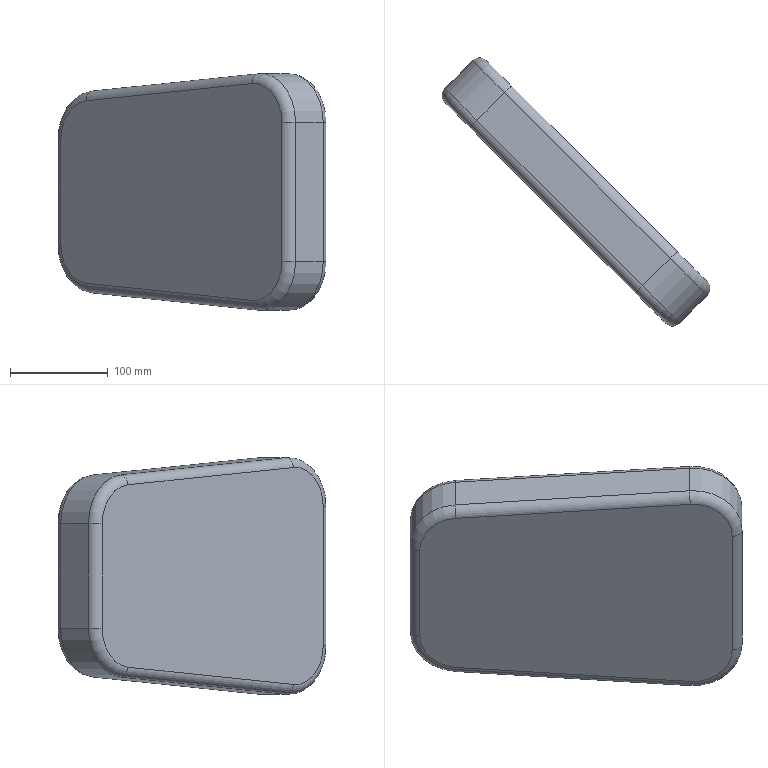Component | NX | SEAT_CUSH | 1 solid | 26 faces | volume 4415373 mm3 | cylinder 12 | torus 8 | plane 6 | commonest cylinder face diameters 20 x8 100 x4